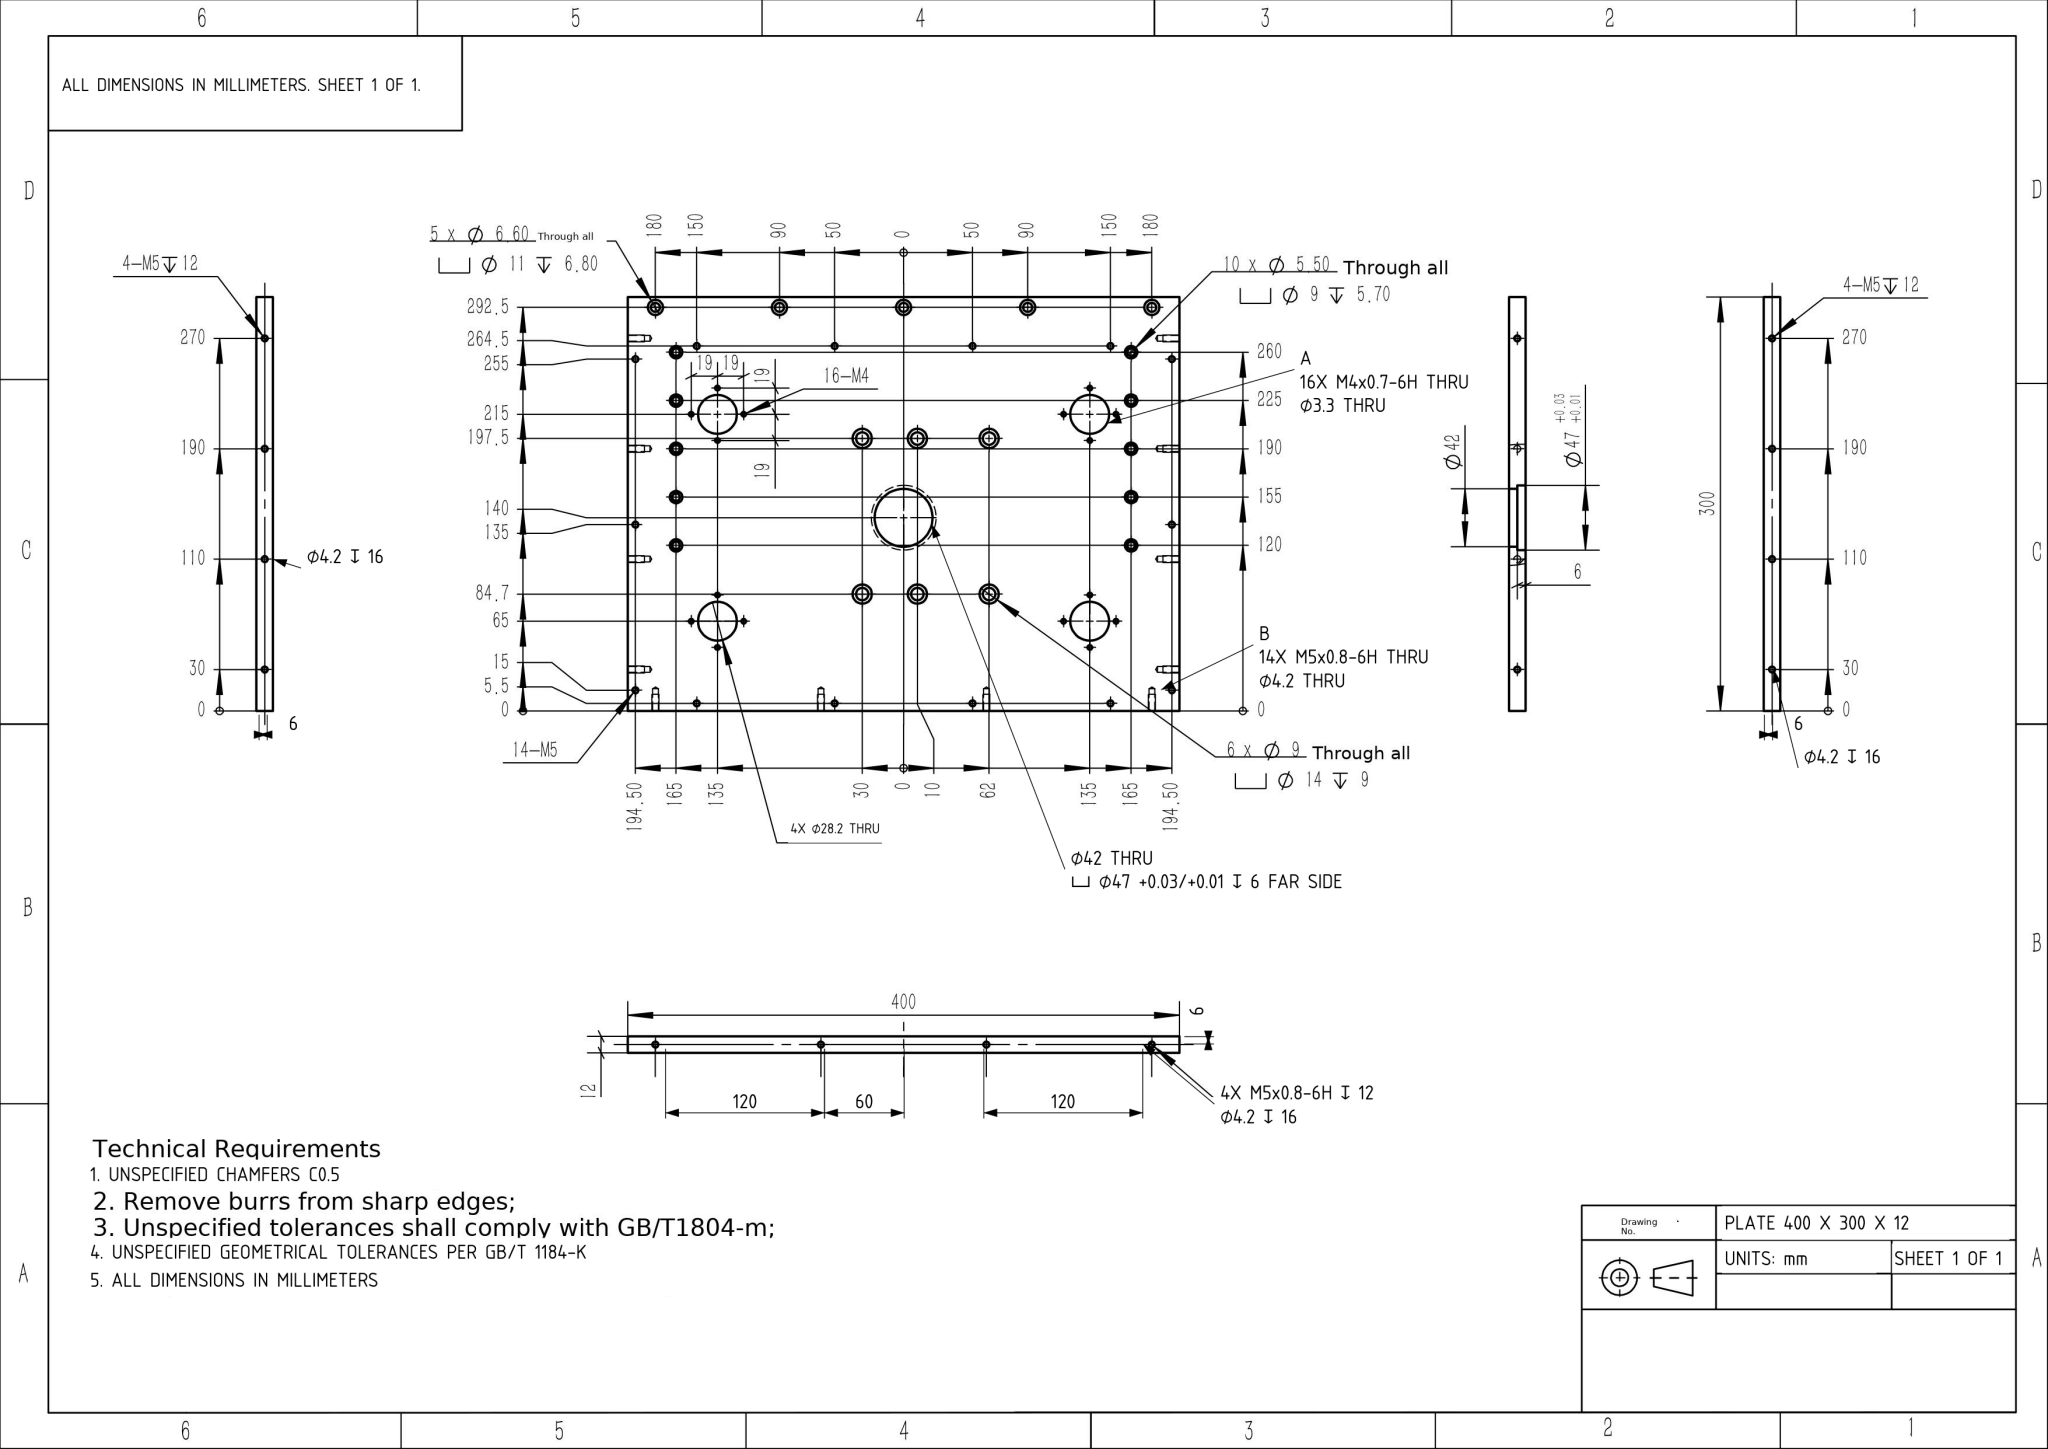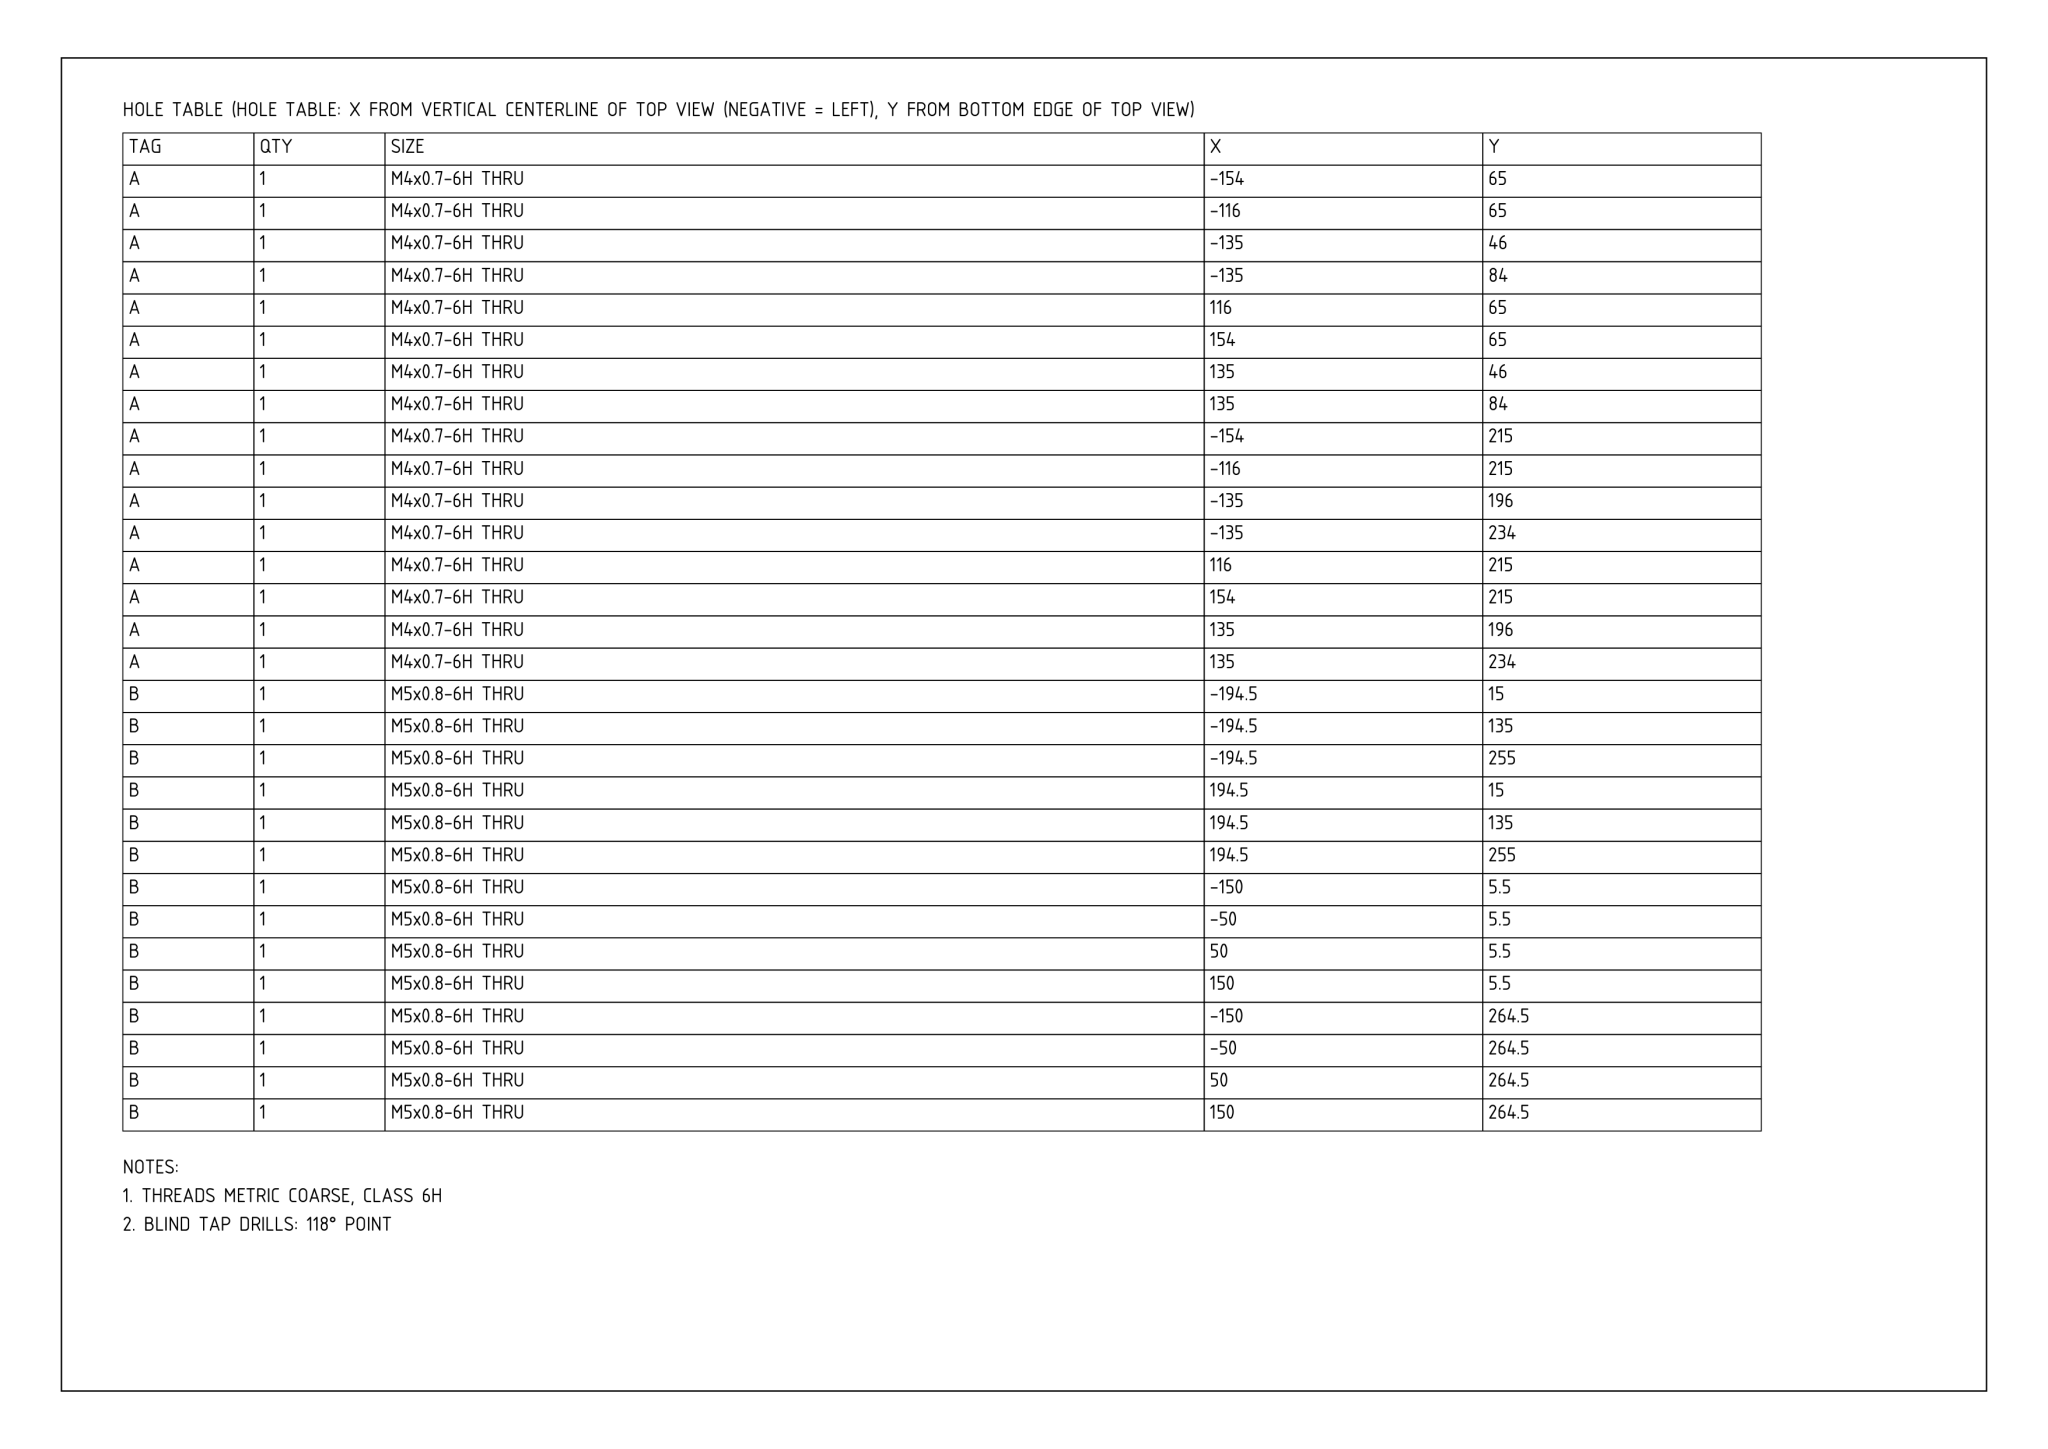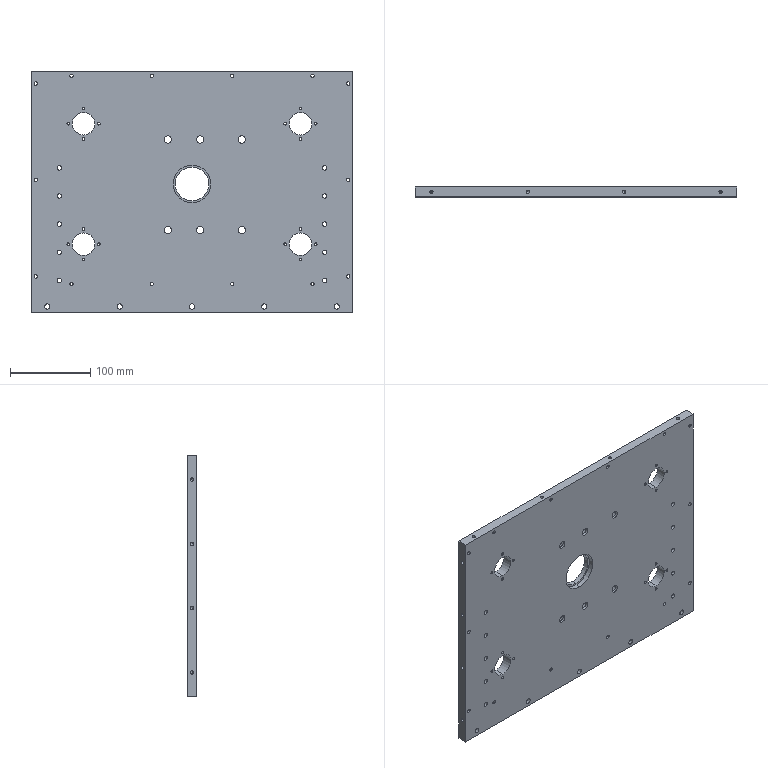Part | NX | mm | 1 solid | 232 faces | box 400 x 12 x 300 mm | volume 1365897 mm3 | cylinder 180 | plane 28 | cone 24 | commonest cylinder face diameters 4.2 x52 9 x32 3.3 x32 5.5 x20 14 x12 11 x10 6.6 x10 28.2 x8